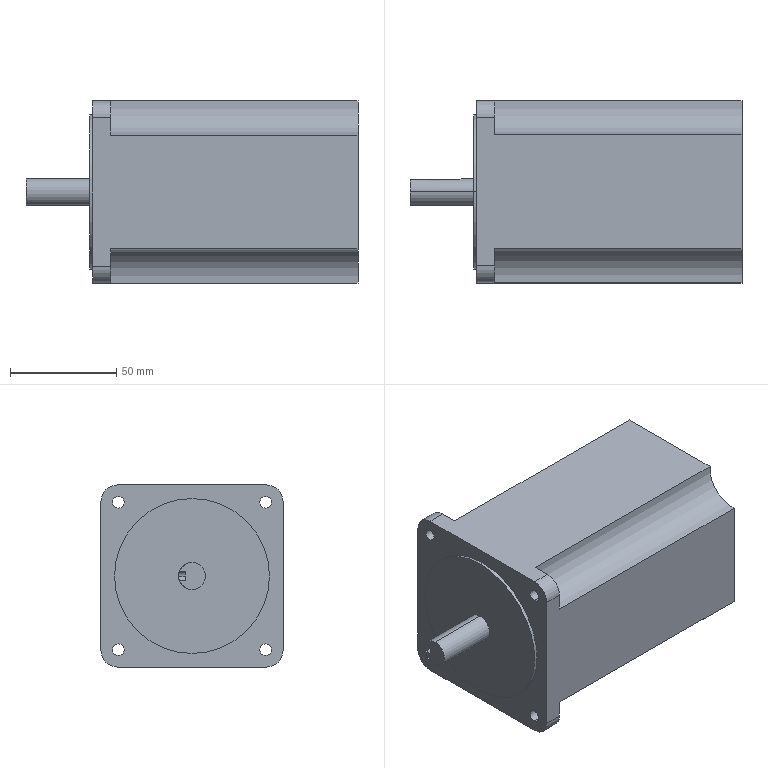Component | SolidWorks | StepperMotor86J18118-842-1 | 1 solid | 39 faces | volume 831525 mm3 | cylinder 24 | plane 15 | commonest cylinder face diameters 5.5 x8 30 x6 16 x4 12.7 x2 73 x2 4 x2